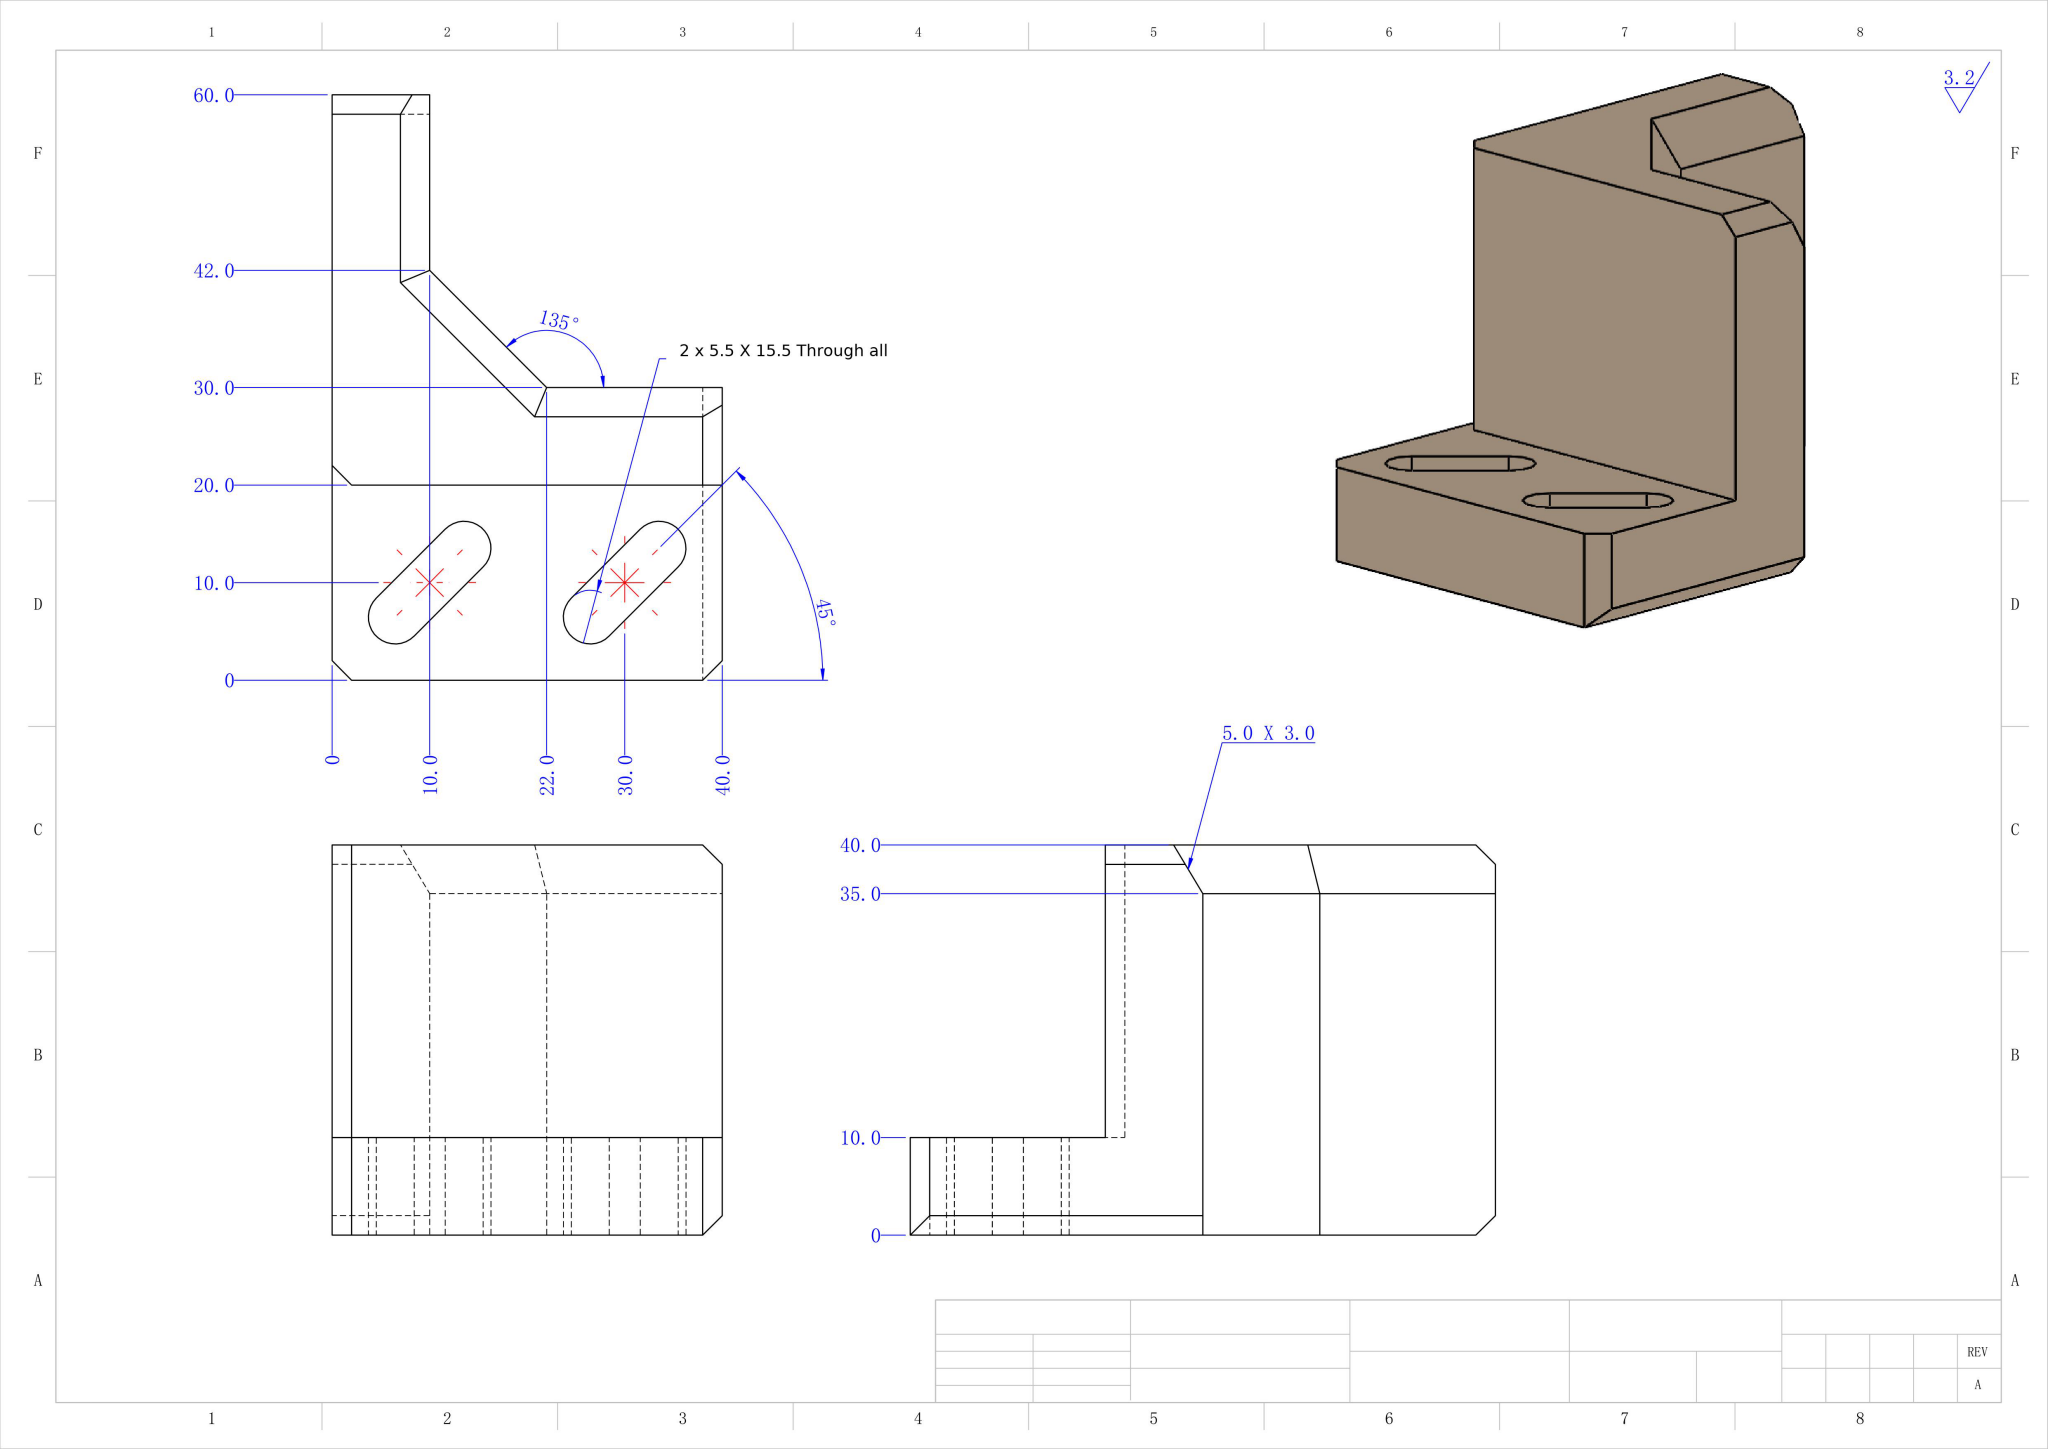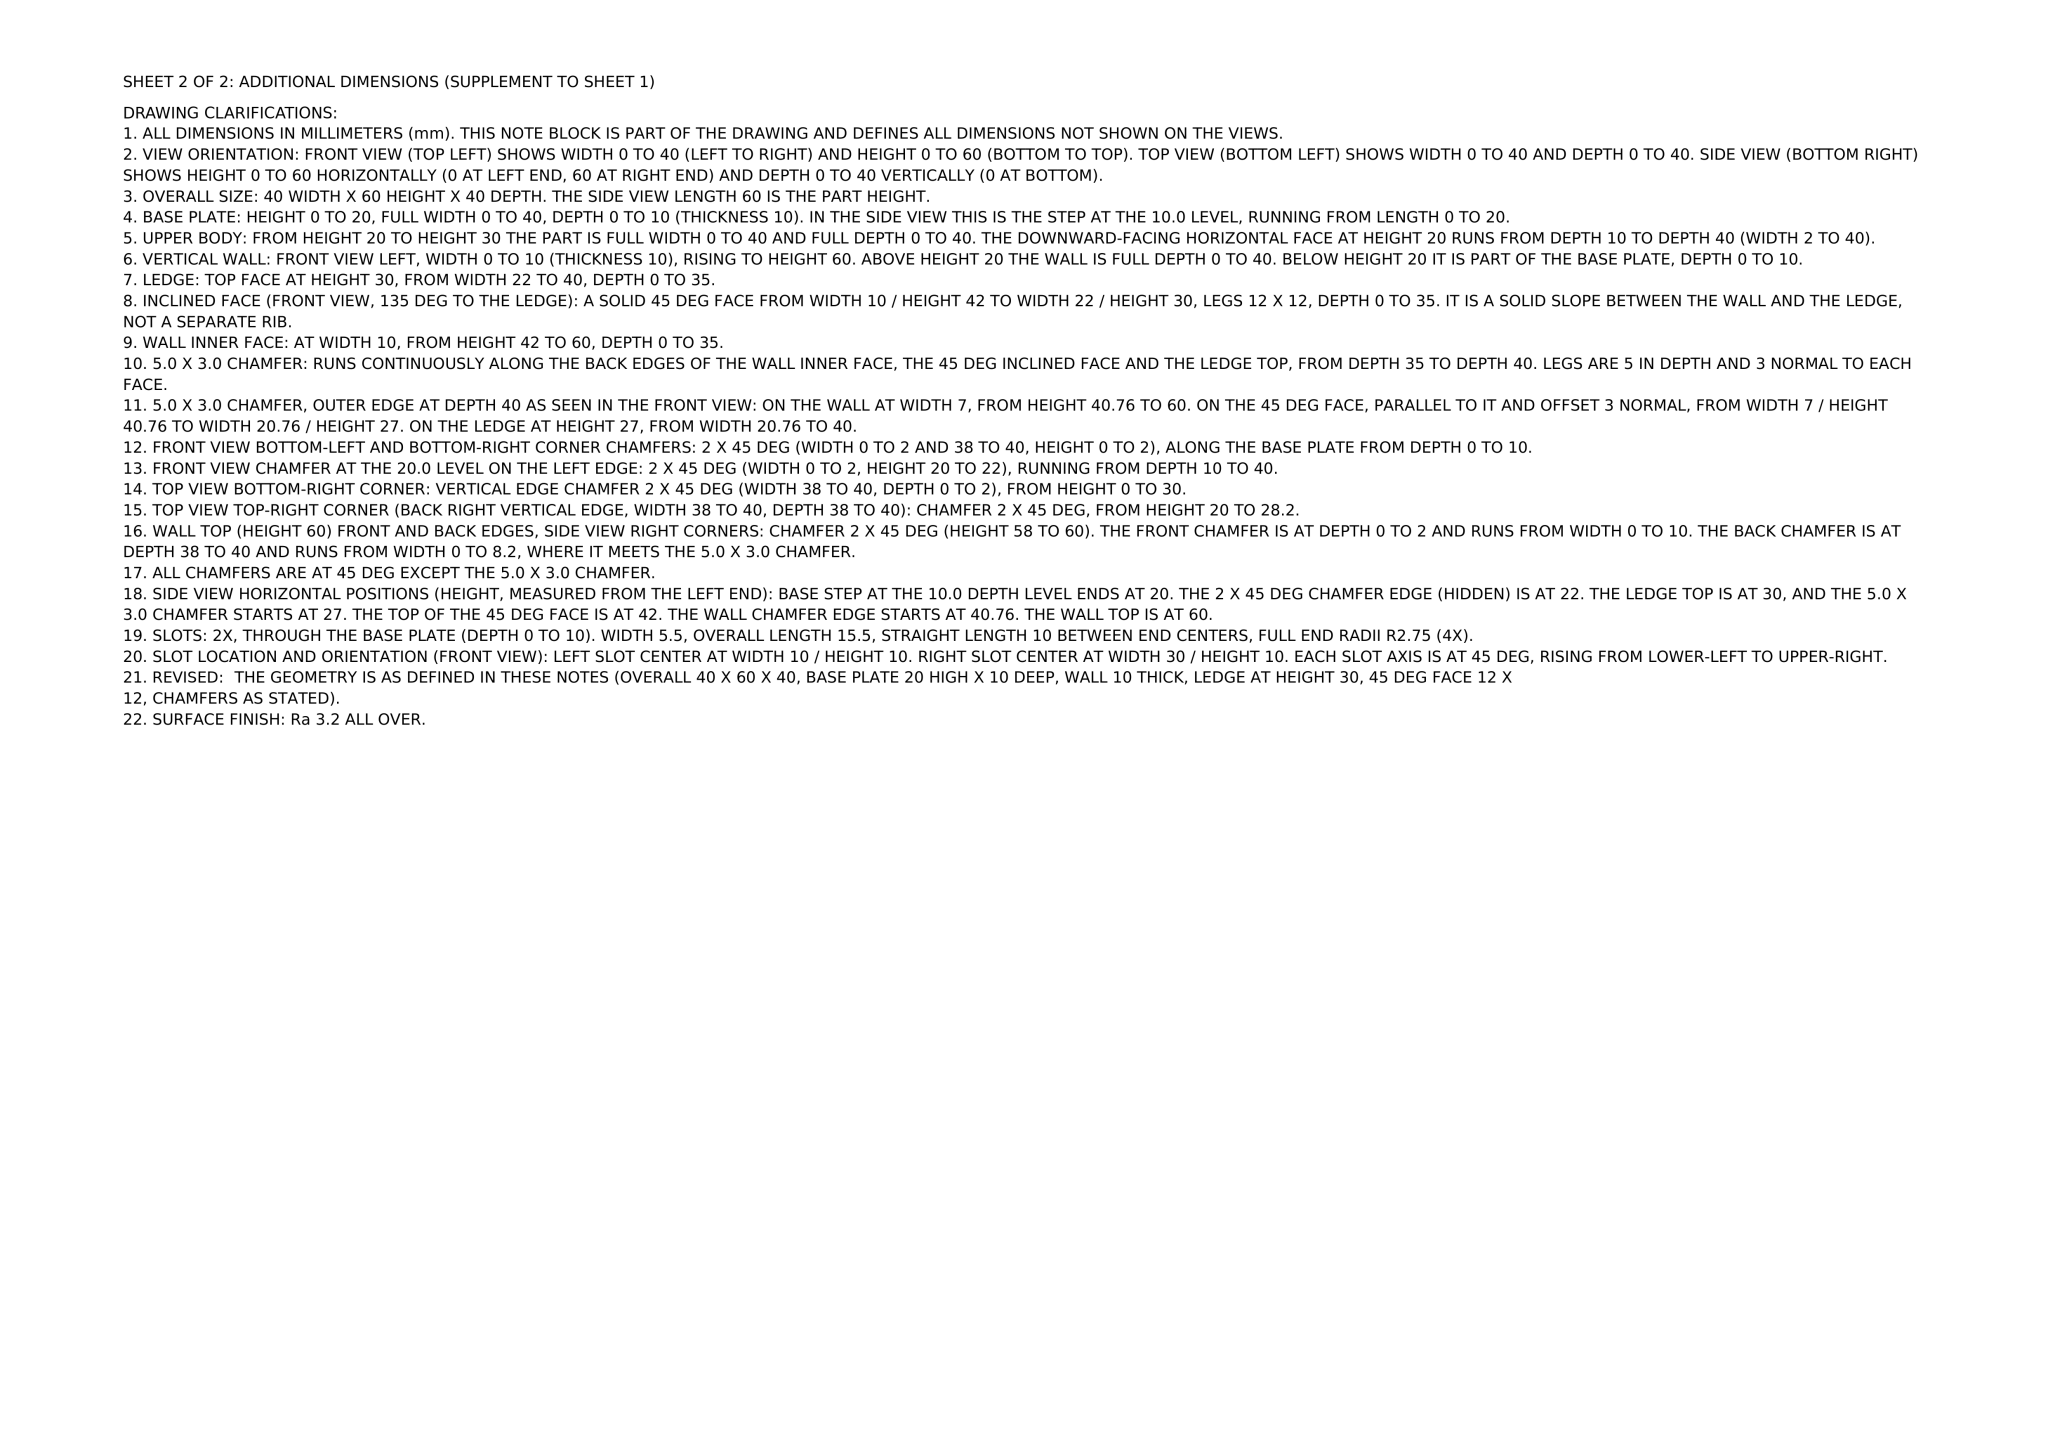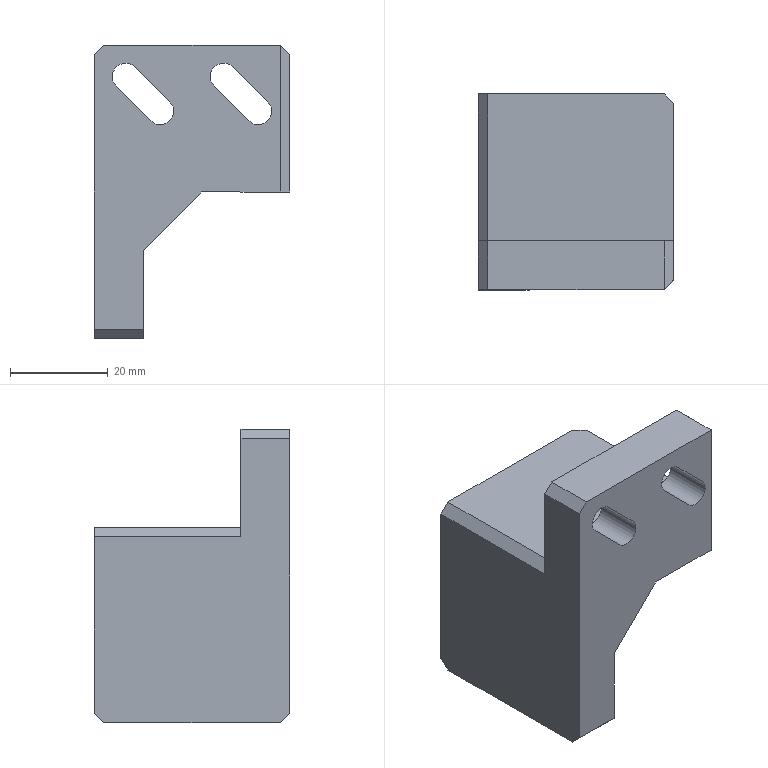Part | NX | mm | 1 solid | 31 faces | box 40 x 40 x 60 mm | volume 36688 mm3 | plane 25 | cylinder 6 | commonest cylinder face diameters 5.5 x6